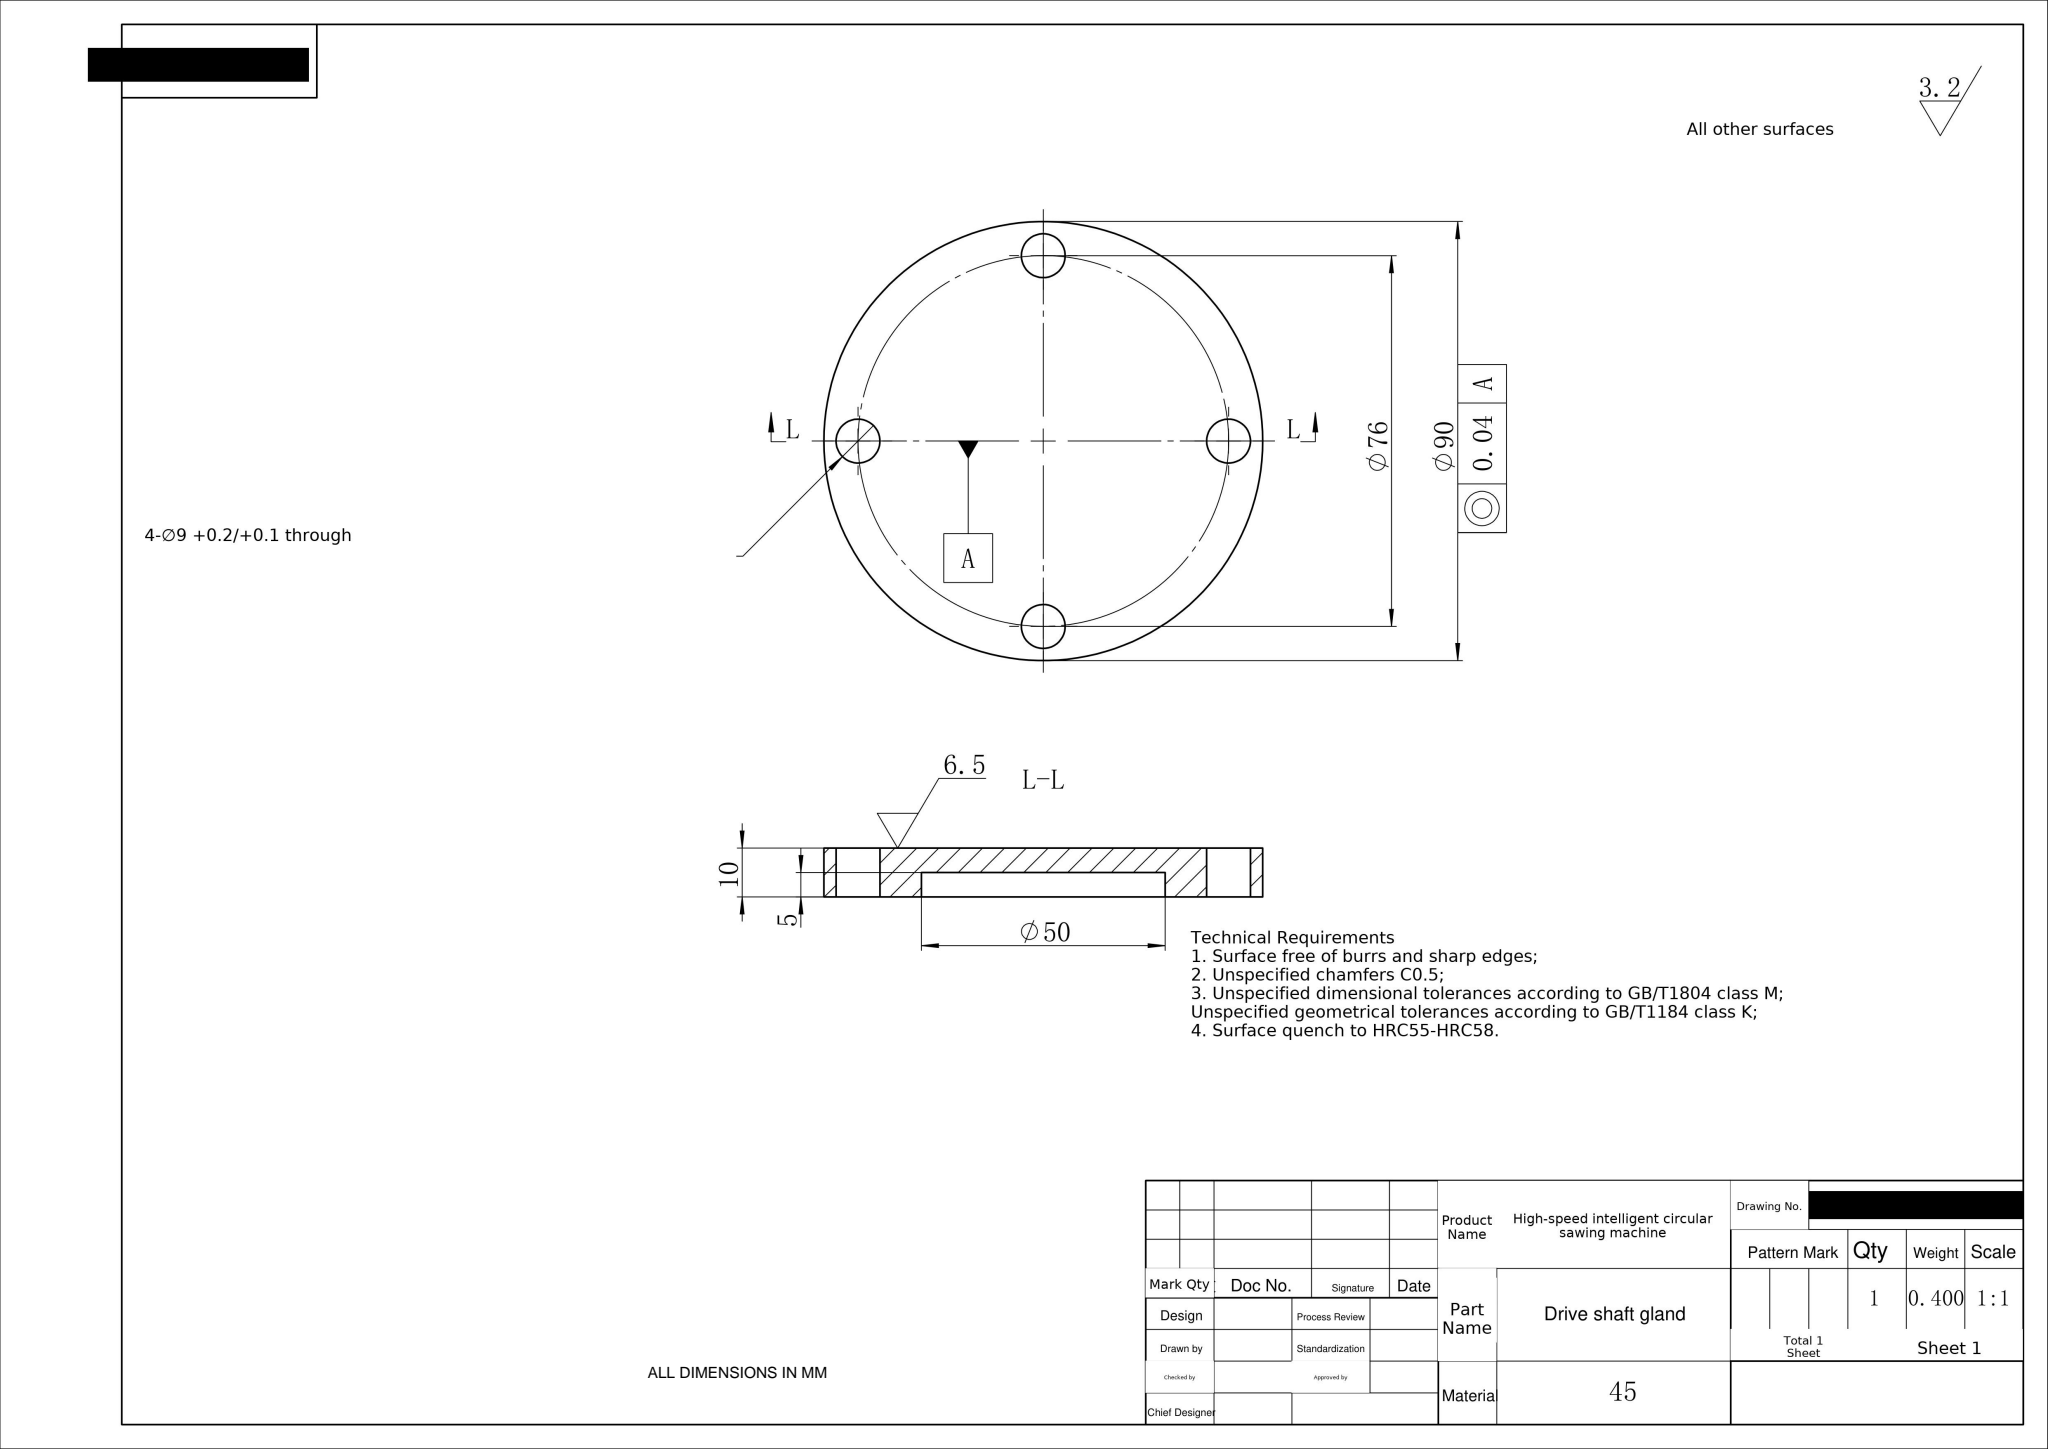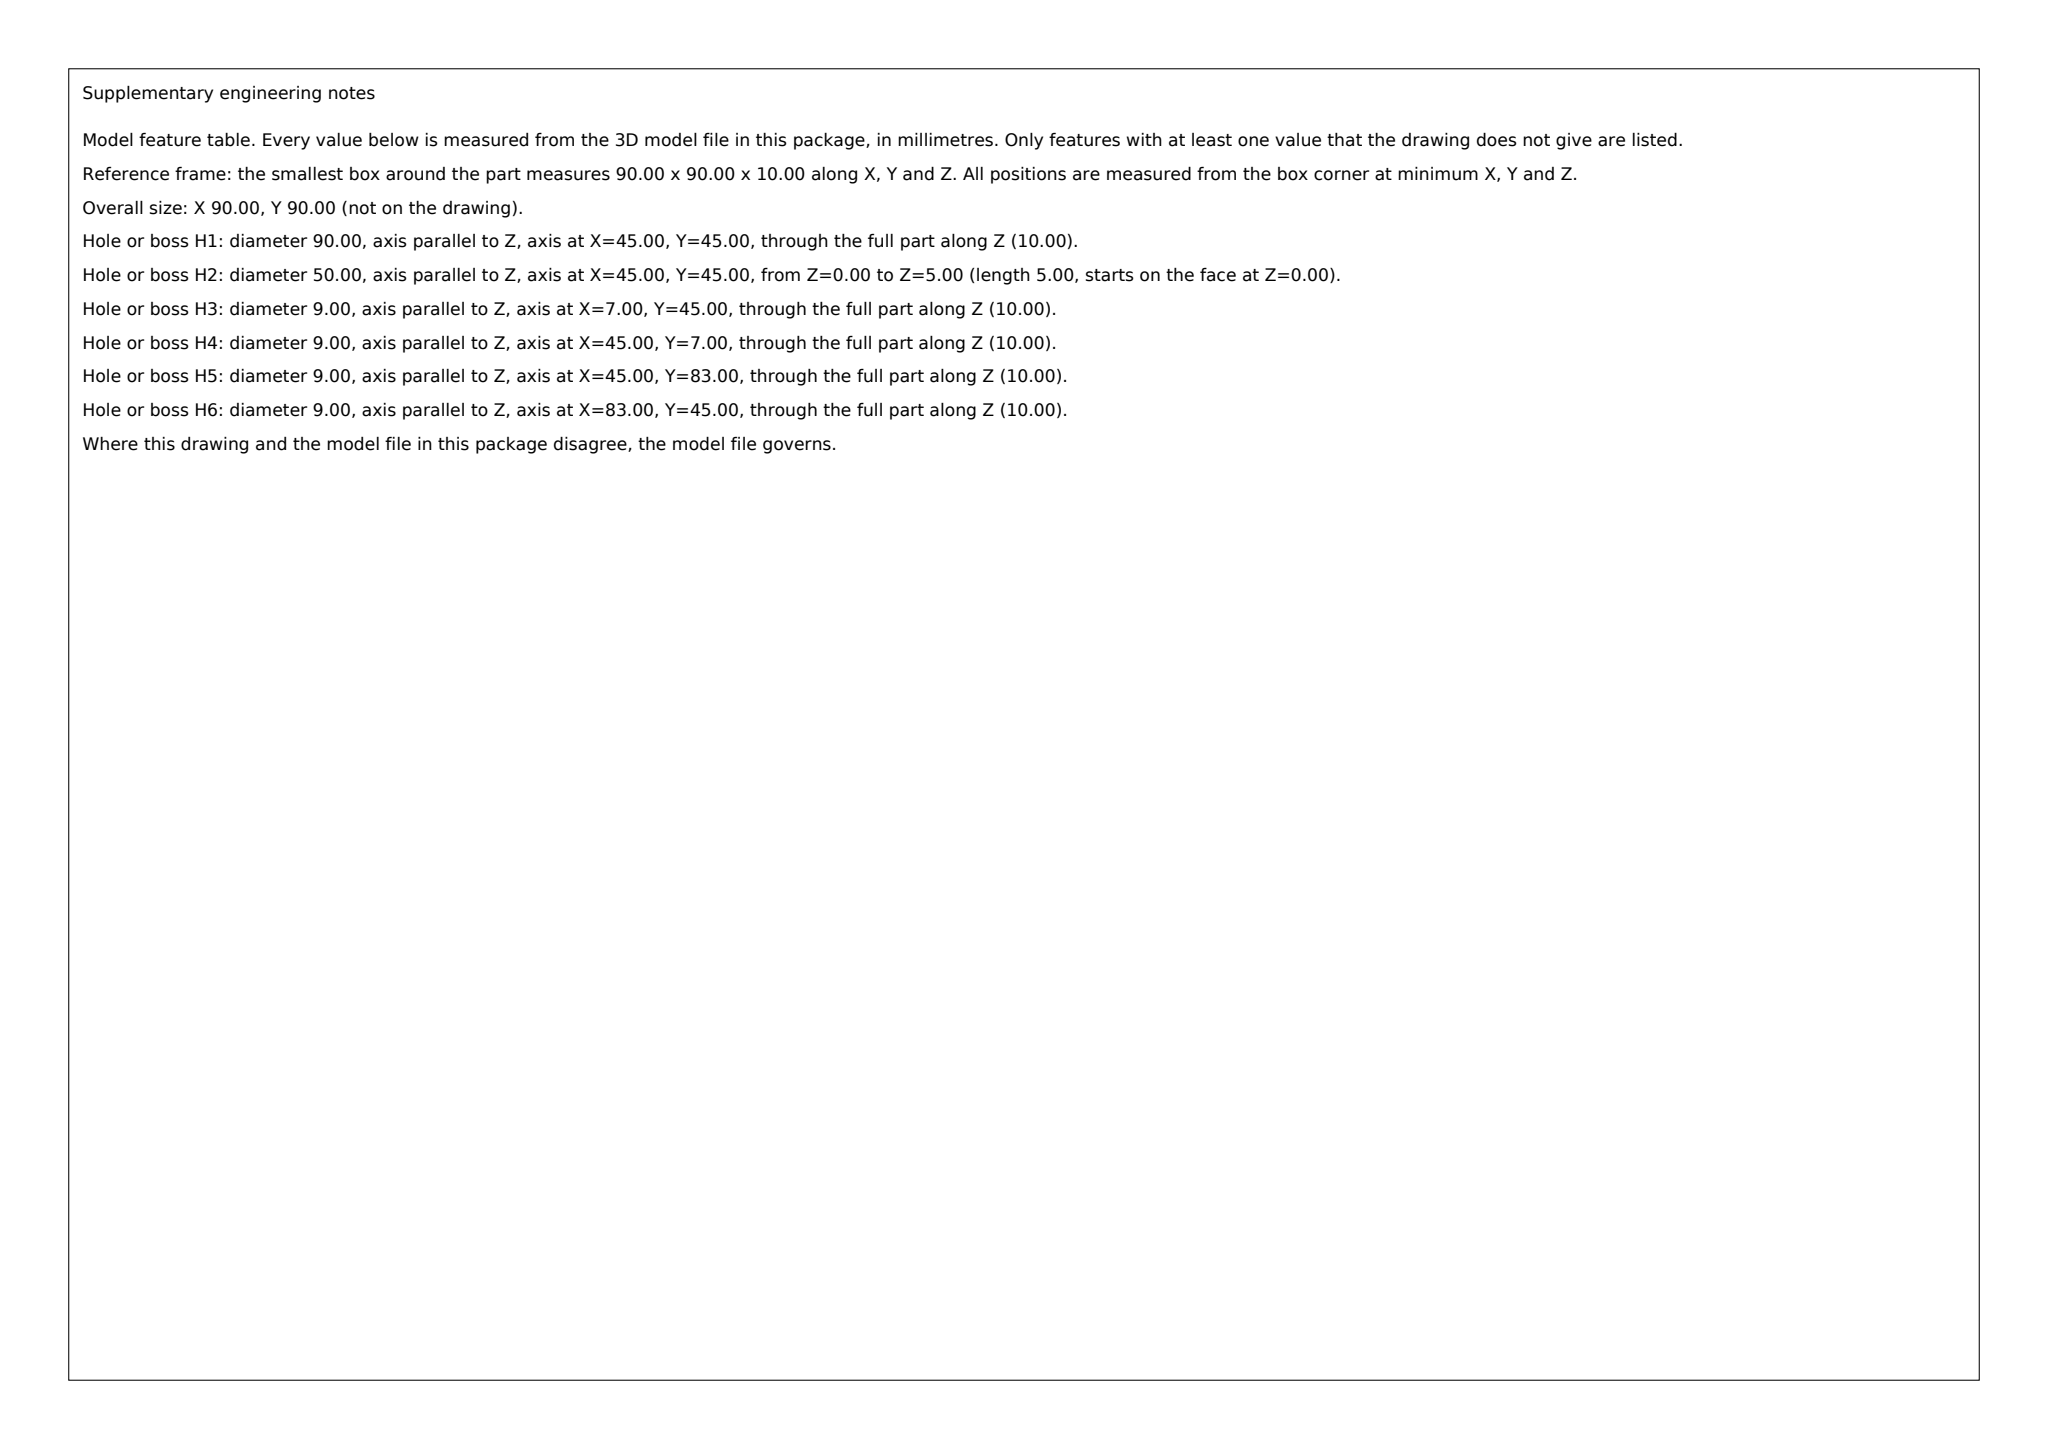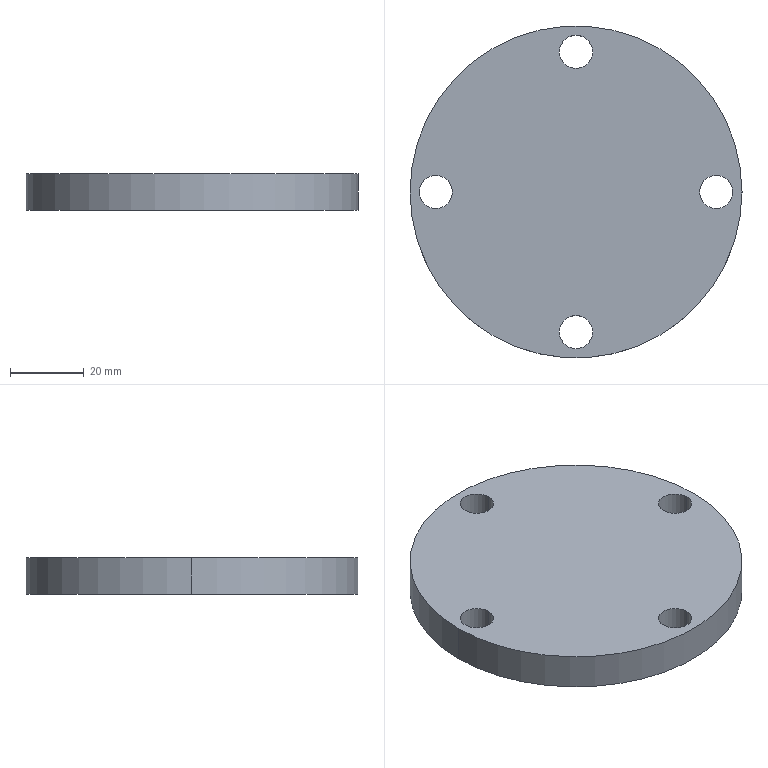Part | SolidWorks | mm | material 45 | 1 solid | 15 faces | box 90 x 90 x 10 mm | volume 51255 mm3 | cylinder 12 | plane 3 | commonest cylinder face diameters 9 x8 50 x2 90 x2
build123d program:
from build123d import *

# Parameters (mm, degrees)
SKETCH1_R           = 45
BOSS_EXTRUDE1_DEPTH = 10
SKETCH4_R           = 4.5
CUT_EXTRUDE2_DEPTH  = 65.42
SKETCH2_R           = 25
CUT_EXTRUDE3_DEPTH  = 5


with BuildPart() as part:
    # Sketch1 → Boss-Extrude1 (new body)
    with BuildSketch(Plane.XY):
        Circle(SKETCH1_R)
    extrude(amount=BOSS_EXTRUDE1_DEPTH)

    # Sketch4 → Cut-Extrude2 (cut, through all)
    with BuildSketch(Plane(origin=(0, 0, 0), x_dir=(-1, 0, 0), z_dir=(0, 0, -1))):
        with Locations((0, -38)):
            Circle(SKETCH4_R)
        with Locations((38, 0)):
            Circle(SKETCH4_R)
        with Locations((0, 38)):
            Circle(SKETCH4_R)
        with Locations((-38, 0)):
            Circle(SKETCH4_R)
    extrude(amount=-CUT_EXTRUDE2_DEPTH, mode=Mode.SUBTRACT)

    # Sketch2 → Cut-Extrude3 (cut)
    with BuildSketch(Plane(origin=(0, 0, 0), x_dir=(-1, 0, 0), z_dir=(0, 0, -1))):
        Circle(SKETCH2_R)
    extrude(amount=-CUT_EXTRUDE3_DEPTH, mode=Mode.SUBTRACT)


solid = part.part
STEP:
#1=CARTESIAN_POINT('',(25.,0.,5.));
#2=VERTEX_POINT('',#1);
#3=CARTESIAN_POINT('',(-25.,0.,5.));
#4=VERTEX_POINT('',#3);
#5=CARTESIAN_POINT('',(0.,0.,5.));
#6=DIRECTION('',(0.,0.,-1.));
#7=DIRECTION('',(-1.,0.,0.));
#8=AXIS2_PLACEMENT_3D('',#5,#6,#7);
#9=CIRCLE('',#8,25.);
#10=EDGE_CURVE('',#2,#4,#9,.T.);
#11=ORIENTED_EDGE('',*,*,#10,.F.);
#12=CARTESIAN_POINT('',(25.,0.,0.));
#13=VERTEX_POINT('',#12);
#14=CARTESIAN_POINT('',(25.,0.,5.));
#15=DIRECTION('',(0.,0.,-1.));
#16=VECTOR('',#15,1000.);
#17=LINE('',#14,#16);
#18=EDGE_CURVE('',#2,#13,#17,.T.);
#19=ORIENTED_EDGE('',*,*,#18,.T.);
#20=CARTESIAN_POINT('',(-25.,0.,0.));
#21=VERTEX_POINT('',#20);
#22=CARTESIAN_POINT('',(0.,0.,0.));
#23=DIRECTION('',(0.,0.,-1.));
#24=DIRECTION('',(-1.,0.,0.));
#25=AXIS2_PLACEMENT_3D('',#22,#23,#24);
#26=CIRCLE('',#25,25.);
#27=EDGE_CURVE('',#13,#21,#26,.T.);
#28=ORIENTED_EDGE('',*,*,#27,.T.);
#29=CARTESIAN_POINT('',(-25.,0.,5.));
#30=DIRECTION('',(0.,0.,-1.));
#31=VECTOR('',#30,1000.);
#32=LINE('',#29,#31);
#33=EDGE_CURVE('',#4,#21,#32,.T.);
#34=ORIENTED_EDGE('',*,*,#33,.F.);
#35=EDGE_LOOP('',(#11,#19,#28,#34));
#36=FACE_OUTER_BOUND('',#35,.T.);
#37=CARTESIAN_POINT('',(0.,0.,5.));
#38=DIRECTION('',(0.,0.,-1.));
#39=DIRECTION('',(-1.,0.,0.));
#40=AXIS2_PLACEMENT_3D('',#37,#38,#39);
#41=CYLINDRICAL_SURFACE('',#40,25.);
#42=ADVANCED_FACE('',(#36),#41,.F.);
#43=CARTESIAN_POINT('',(42.5,0.,10.));
#44=VERTEX_POINT('',#43);
#45=CARTESIAN_POINT('',(33.5,0.,10.));
#46=VERTEX_POINT('',#45);
#47=CARTESIAN_POINT('',(38.,0.,10.));
#48=DIRECTION('',(0.,0.,-1.));
#49=DIRECTION('',(-1.,0.,0.));
#50=AXIS2_PLACEMENT_3D('',#47,#48,#49);
#51=CIRCLE('',#50,4.5);
#52=EDGE_CURVE('',#44,#46,#51,.T.);
#53=ORIENTED_EDGE('',*,*,#52,.F.);
#54=CARTESIAN_POINT('',(42.5,0.,0.));
#55=VERTEX_POINT('',#54);
#56=CARTESIAN_POINT('',(42.5,0.,10.));
#57=DIRECTION('',(0.,0.,-1.));
#58=VECTOR('',#57,1000.);
#59=LINE('',#56,#58);
#60=EDGE_CURVE('',#44,#55,#59,.T.);
#61=ORIENTED_EDGE('',*,*,#60,.T.);
#62=CARTESIAN_POINT('',(33.5,0.,0.));
#63=VERTEX_POINT('',#62);
#64=CARTESIAN_POINT('',(38.,0.,0.));
#65=DIRECTION('',(0.,0.,-1.));
#66=DIRECTION('',(-1.,0.,0.));
#67=AXIS2_PLACEMENT_3D('',#64,#65,#66);
#68=CIRCLE('',#67,4.5);
#69=EDGE_CURVE('',#55,#63,#68,.T.);
#70=ORIENTED_EDGE('',*,*,#69,.T.);
#71=CARTESIAN_POINT('',(33.5,0.,10.));
#72=DIRECTION('',(0.,0.,-1.));
#73=VECTOR('',#72,1000.);
#74=LINE('',#71,#73);
#75=EDGE_CURVE('',#46,#63,#74,.T.);
#76=ORIENTED_EDGE('',*,*,#75,.F.);
#77=EDGE_LOOP('',(#53,#61,#70,#76));
#78=FACE_OUTER_BOUND('',#77,.T.);
#79=CARTESIAN_POINT('',(38.,0.,10.));
#80=DIRECTION('',(0.,0.,-1.));
#81=DIRECTION('',(-1.,0.,0.));
#82=AXIS2_PLACEMENT_3D('',#79,#80,#81);
#83=CYLINDRICAL_SURFACE('',#82,4.5);
#84=ADVANCED_FACE('',(#78),#83,.F.);
#85=CARTESIAN_POINT('',(4.5,38.,10.));
#86=VERTEX_POINT('',#85);
#87=CARTESIAN_POINT('',(-4.5,38.,10.));
#88=VERTEX_POINT('',#87);
#89=CARTESIAN_POINT('',(0.,38.,10.));
#90=DIRECTION('',(0.,0.,-1.));
#91=DIRECTION('',(-1.,0.,0.));
#92=AXIS2_PLACEMENT_3D('',#89,#90,#91);
#93=CIRCLE('',#92,4.5);
#94=EDGE_CURVE('',#86,#88,#93,.T.);
#95=ORIENTED_EDGE('',*,*,#94,.F.);
#96=CARTESIAN_POINT('',(4.5,38.,0.));
#97=VERTEX_POINT('',#96);
#98=CARTESIAN_POINT('',(4.5,38.,10.));
#99=DIRECTION('',(0.,0.,-1.));
#100=VECTOR('',#99,1000.);
#101=LINE('',#98,#100);
#102=EDGE_CURVE('',#86,#97,#101,.T.);
#103=ORIENTED_EDGE('',*,*,#102,.T.);
#104=CARTESIAN_POINT('',(-4.5,38.,0.));
#105=VERTEX_POINT('',#104);
#106=CARTESIAN_POINT('',(0.,38.,0.));
#107=DIRECTION('',(0.,0.,-1.));
#108=DIRECTION('',(-1.,0.,0.));
#109=AXIS2_PLACEMENT_3D('',#106,#107,#108);
#110=CIRCLE('',#109,4.5);
#111=EDGE_CURVE('',#97,#105,#110,.T.);
#112=ORIENTED_EDGE('',*,*,#111,.T.);
#113=CARTESIAN_POINT('',(-4.5,38.,10.));
#114=DIRECTION('',(0.,0.,-1.));
#115=VECTOR('',#114,1000.);
#116=LINE('',#113,#115);
#117=EDGE_CURVE('',#88,#105,#116,.T.);
#118=ORIENTED_EDGE('',*,*,#117,.F.);
#119=EDGE_LOOP('',(#95,#103,#112,#118));
#120=FACE_OUTER_BOUND('',#119,.T.);
#121=CARTESIAN_POINT('',(0.,38.,10.));
#122=DIRECTION('',(0.,0.,-1.));
#123=DIRECTION('',(-1.,0.,0.));
#124=AXIS2_PLACEMENT_3D('',#121,#122,#123);
#125=CYLINDRICAL_SURFACE('',#124,4.5);
#126=ADVANCED_FACE('',(#120),#125,.F.);
#127=CARTESIAN_POINT('',(-33.5,0.,10.));
#128=VERTEX_POINT('',#127);
#129=CARTESIAN_POINT('',(-42.5,0.,10.));
#130=VERTEX_POINT('',#129);
#131=CARTESIAN_POINT('',(-38.,0.,10.));
#132=DIRECTION('',(0.,0.,-1.));
#133=DIRECTION('',(-1.,0.,0.));
#134=AXIS2_PLACEMENT_3D('',#131,#132,#133);
#135=CIRCLE('',#134,4.5);
#136=EDGE_CURVE('',#128,#130,#135,.T.);
#137=ORIENTED_EDGE('',*,*,#136,.F.);
#138=CARTESIAN_POINT('',(-33.5,0.,0.));
#139=VERTEX_POINT('',#138);
#140=CARTESIAN_POINT('',(-33.5,0.,10.));
#141=DIRECTION('',(0.,0.,-1.));
#142=VECTOR('',#141,1000.);
#143=LINE('',#140,#142);
#144=EDGE_CURVE('',#128,#139,#143,.T.);
#145=ORIENTED_EDGE('',*,*,#144,.T.);
#146=CARTESIAN_POINT('',(-42.5,0.,0.));
#147=VERTEX_POINT('',#146);
#148=CARTESIAN_POINT('',(-38.,0.,0.));
#149=DIRECTION('',(0.,0.,-1.));
#150=DIRECTION('',(-1.,0.,0.));
#151=AXIS2_PLACEMENT_3D('',#148,#149,#150);
#152=CIRCLE('',#151,4.5);
#153=EDGE_CURVE('',#139,#147,#152,.T.);
#154=ORIENTED_EDGE('',*,*,#153,.T.);
#155=CARTESIAN_POINT('',(-42.5,0.,10.));
#156=DIRECTION('',(0.,0.,-1.));
#157=VECTOR('',#156,1000.);
#158=LINE('',#155,#157);
#159=EDGE_CURVE('',#130,#147,#158,.T.);
#160=ORIENTED_EDGE('',*,*,#159,.F.);
#161=EDGE_LOOP('',(#137,#145,#154,#160));
#162=FACE_OUTER_BOUND('',#161,.T.);
#163=CARTESIAN_POINT('',(-38.,0.,10.));
#164=DIRECTION('',(0.,0.,-1.));
#165=DIRECTION('',(-1.,0.,0.));
#166=AXIS2_PLACEMENT_3D('',#163,#164,#165);
#167=CYLINDRICAL_SURFACE('',#166,4.5);
#168=ADVANCED_FACE('',(#162),#167,.F.);
#169=CARTESIAN_POINT('',(4.5,-38.,10.));
#170=VERTEX_POINT('',#169);
#171=CARTESIAN_POINT('',(-4.5,-38.,10.));
#172=VERTEX_POINT('',#171);
#173=CARTESIAN_POINT('',(0.,-38.,10.));
#174=DIRECTION('',(0.,0.,-1.));
#175=DIRECTION('',(-1.,0.,0.));
#176=AXIS2_PLACEMENT_3D('',#173,#174,#175);
#177=CIRCLE('',#176,4.5);
#178=EDGE_CURVE('',#170,#172,#177,.T.);
#179=ORIENTED_EDGE('',*,*,#178,.F.);
#180=CARTESIAN_POINT('',(4.5,-38.,0.));
#181=VERTEX_POINT('',#180);
#182=CARTESIAN_POINT('',(4.5,-38.,10.));
#183=DIRECTION('',(0.,0.,-1.));
#184=VECTOR('',#183,1000.);
#185=LINE('',#182,#184);
#186=EDGE_CURVE('',#170,#181,#185,.T.);
#187=ORIENTED_EDGE('',*,*,#186,.T.);
#188=CARTESIAN_POINT('',(-4.5,-38.,0.));
#189=VERTEX_POINT('',#188);
#190=CARTESIAN_POINT('',(0.,-38.,0.));
#191=DIRECTION('',(0.,0.,-1.));
#192=DIRECTION('',(-1.,0.,0.));
#193=AXIS2_PLACEMENT_3D('',#190,#191,#192);
#194=CIRCLE('',#193,4.5);
#195=EDGE_CURVE('',#181,#189,#194,.T.);
#196=ORIENTED_EDGE('',*,*,#195,.T.);
#197=CARTESIAN_POINT('',(-4.5,-38.,10.));
#198=DIRECTION('',(0.,0.,-1.));
#199=VECTOR('',#198,1000.);
#200=LINE('',#197,#199);
#201=EDGE_CURVE('',#172,#189,#200,.T.);
#202=ORIENTED_EDGE('',*,*,#201,.F.);
#203=EDGE_LOOP('',(#179,#187,#196,#202));
#204=FACE_OUTER_BOUND('',#203,.T.);
#205=CARTESIAN_POINT('',(0.,-38.,10.));
#206=DIRECTION('',(0.,0.,-1.));
#207=DIRECTION('',(-1.,0.,0.));
#208=AXIS2_PLACEMENT_3D('',#205,#206,#207);
#209=CYLINDRICAL_SURFACE('',#208,4.5);
#210=ADVANCED_FACE('',(#204),#209,.F.);
#211=CARTESIAN_POINT('',(45.,0.,10.));
#212=VERTEX_POINT('',#211);
#213=CARTESIAN_POINT('',(-45.,0.,10.));
#214=VERTEX_POINT('',#213);
#215=CARTESIAN_POINT('',(0.,0.,10.));
#216=DIRECTION('',(0.,0.,1.));
#217=DIRECTION('',(1.,0.,0.));
#218=AXIS2_PLACEMENT_3D('',#215,#216,#217);
#219=CIRCLE('',#218,45.);
#220=EDGE_CURVE('',#212,#214,#219,.T.);
#221=ORIENTED_EDGE('',*,*,#220,.F.);
#222=CARTESIAN_POINT('',(45.,0.,0.));
#223=VERTEX_POINT('',#222);
#224=CARTESIAN_POINT('',(45.,0.,10.));
#225=DIRECTION('',(0.,0.,-1.));
#226=VECTOR('',#225,1000.);
#227=LINE('',#224,#226);
#228=EDGE_CURVE('',#212,#223,#227,.T.);
#229=ORIENTED_EDGE('',*,*,#228,.T.);
#230=CARTESIAN_POINT('',(-45.,0.,0.));
#231=VERTEX_POINT('',#230);
#232=CARTESIAN_POINT('',(0.,0.,0.));
#233=DIRECTION('',(0.,0.,1.));
#234=DIRECTION('',(1.,0.,0.));
#235=AXIS2_PLACEMENT_3D('',#232,#233,#234);
#236=CIRCLE('',#235,45.);
#237=EDGE_CURVE('',#223,#231,#236,.T.);
#238=ORIENTED_EDGE('',*,*,#237,.T.);
#239=CARTESIAN_POINT('',(-45.,0.,10.));
#240=DIRECTION('',(0.,0.,-1.));
#241=VECTOR('',#240,1000.);
#242=LINE('',#239,#241);
#243=EDGE_CURVE('',#214,#231,#242,.T.);
#244=ORIENTED_EDGE('',*,*,#243,.F.);
#245=EDGE_LOOP('',(#221,#229,#238,#244));
#246=FACE_OUTER_BOUND('',#245,.T.);
#247=CARTESIAN_POINT('',(0.,0.,10.));
#248=DIRECTION('',(0.,0.,-1.));
#249=DIRECTION('',(-1.,0.,0.));
#250=AXIS2_PLACEMENT_3D('',#247,#248,#249);
#251=CYLINDRICAL_SURFACE('',#250,45.);
#252=ADVANCED_FACE('',(#246),#251,.T.);
#253=ORIENTED_EDGE('',*,*,#228,.F.);
#254=CARTESIAN_POINT('',(0.,0.,10.));
#255=DIRECTION('',(0.,0.,1.));
#256=DIRECTION('',(1.,0.,0.));
#257=AXIS2_PLACEMENT_3D('',#254,#255,#256);
#258=CIRCLE('',#257,45.);
#259=EDGE_CURVE('',#214,#212,#258,.T.);
#260=ORIENTED_EDGE('',*,*,#259,.F.);
#261=ORIENTED_EDGE('',*,*,#243,.T.);
#262=CARTESIAN_POINT('',(0.,0.,0.));
#263=DIRECTION('',(0.,0.,1.));
#264=DIRECTION('',(1.,0.,0.));
#265=AXIS2_PLACEMENT_3D('',#262,#263,#264);
#266=CIRCLE('',#265,45.);
#267=EDGE_CURVE('',#231,#223,#266,.T.);
#268=ORIENTED_EDGE('',*,*,#267,.T.);
#269=EDGE_LOOP('',(#253,#260,#261,#268));
#270=FACE_OUTER_BOUND('',#269,.T.);
#271=CARTESIAN_POINT('',(0.,0.,10.));
#272=DIRECTION('',(0.,0.,-1.));
#273=DIRECTION('',(-1.,0.,0.));
#274=AXIS2_PLACEMENT_3D('',#271,#272,#273);
#275=CYLINDRICAL_SURFACE('',#274,45.);
#276=ADVANCED_FACE('',(#270),#275,.T.);
#277=CARTESIAN_POINT('',(38.,0.,10.));
#278=DIRECTION('',(0.,0.,-1.));
#279=DIRECTION('',(-1.,0.,0.));
#280=AXIS2_PLACEMENT_3D('',#277,#278,#279);
#281=CIRCLE('',#280,4.5);
#282=EDGE_CURVE('',#46,#44,#281,.T.);
#283=ORIENTED_EDGE('',*,*,#282,.T.);
#284=ORIENTED_EDGE('',*,*,#52,.T.);
#285=EDGE_LOOP('',(#283,#284));
#286=FACE_BOUND('',#285,.T.);
#287=CARTESIAN_POINT('',(0.,38.,10.));
#288=DIRECTION('',(0.,0.,-1.));
#289=DIRECTION('',(-1.,0.,0.));
#290=AXIS2_PLACEMENT_3D('',#287,#288,#289);
#291=CIRCLE('',#290,4.5);
#292=EDGE_CURVE('',#88,#86,#291,.T.);
#293=ORIENTED_EDGE('',*,*,#292,.T.);
#294=ORIENTED_EDGE('',*,*,#94,.T.);
#295=EDGE_LOOP('',(#293,#294));
#296=FACE_BOUND('',#295,.T.);
#297=CARTESIAN_POINT('',(-38.,0.,10.));
#298=DIRECTION('',(0.,0.,-1.));
#299=DIRECTION('',(-1.,0.,0.));
#300=AXIS2_PLACEMENT_3D('',#297,#298,#299);
#301=CIRCLE('',#300,4.5);
#302=EDGE_CURVE('',#130,#128,#301,.T.);
#303=ORIENTED_EDGE('',*,*,#302,.T.);
#304=ORIENTED_EDGE('',*,*,#136,.T.);
#305=EDGE_LOOP('',(#303,#304));
#306=FACE_BOUND('',#305,.T.);
#307=CARTESIAN_POINT('',(0.,-38.,10.));
#308=DIRECTION('',(0.,0.,-1.));
#309=DIRECTION('',(-1.,0.,0.));
#310=AXIS2_PLACEMENT_3D('',#307,#308,#309);
#311=CIRCLE('',#310,4.5);
#312=EDGE_CURVE('',#172,#170,#311,.T.);
#313=ORIENTED_EDGE('',*,*,#312,.T.);
#314=ORIENTED_EDGE('',*,*,#178,.T.);
#315=EDGE_LOOP('',(#313,#314));
#316=FACE_BOUND('',#315,.T.);
#317=ORIENTED_EDGE('',*,*,#259,.T.);
#318=ORIENTED_EDGE('',*,*,#220,.T.);
#319=EDGE_LOOP('',(#317,#318));
#320=FACE_OUTER_BOUND('',#319,.T.);
#321=CARTESIAN_POINT('',(0.,0.,10.));
#322=DIRECTION('',(0.,0.,1.));
#323=DIRECTION('',(1.,0.,0.));
#324=AXIS2_PLACEMENT_3D('',#321,#322,#323);
#325=PLANE('',#324);
#326=ADVANCED_FACE('',(#286,#296,#306,#316,#320),#325,.T.);
#327=CARTESIAN_POINT('',(0.,0.,0.));
#328=DIRECTION('',(0.,0.,-1.));
#329=DIRECTION('',(-1.,0.,0.));
#330=AXIS2_PLACEMENT_3D('',#327,#328,#329);
#331=CIRCLE('',#330,25.);
#332=EDGE_CURVE('',#21,#13,#331,.T.);
#333=ORIENTED_EDGE('',*,*,#332,.F.);
#334=ORIENTED_EDGE('',*,*,#27,.F.);
#335=EDGE_LOOP('',(#333,#334));
#336=FACE_BOUND('',#335,.T.);
#337=CARTESIAN_POINT('',(38.,0.,0.));
#338=DIRECTION('',(0.,0.,-1.));
#339=DIRECTION('',(-1.,0.,0.));
#340=AXIS2_PLACEMENT_3D('',#337,#338,#339);
#341=CIRCLE('',#340,4.5);
#342=EDGE_CURVE('',#63,#55,#341,.T.);
#343=ORIENTED_EDGE('',*,*,#342,.F.);
#344=ORIENTED_EDGE('',*,*,#69,.F.);
#345=EDGE_LOOP('',(#343,#344));
#346=FACE_BOUND('',#345,.T.);
#347=CARTESIAN_POINT('',(0.,38.,0.));
#348=DIRECTION('',(0.,0.,-1.));
#349=DIRECTION('',(-1.,0.,0.));
#350=AXIS2_PLACEMENT_3D('',#347,#348,#349);
#351=CIRCLE('',#350,4.5);
#352=EDGE_CURVE('',#105,#97,#351,.T.);
#353=ORIENTED_EDGE('',*,*,#352,.F.);
#354=ORIENTED_EDGE('',*,*,#111,.F.);
#355=EDGE_LOOP('',(#353,#354));
#356=FACE_BOUND('',#355,.T.);
#357=CARTESIAN_POINT('',(-38.,0.,0.));
#358=DIRECTION('',(0.,0.,-1.));
#359=DIRECTION('',(-1.,0.,0.));
#360=AXIS2_PLACEMENT_3D('',#357,#358,#359);
#361=CIRCLE('',#360,4.5);
#362=EDGE_CURVE('',#147,#139,#361,.T.);
#363=ORIENTED_EDGE('',*,*,#362,.F.);
#364=ORIENTED_EDGE('',*,*,#153,.F.);
#365=EDGE_LOOP('',(#363,#364));
#366=FACE_BOUND('',#365,.T.);
#367=CARTESIAN_POINT('',(0.,-38.,0.));
#368=DIRECTION('',(0.,0.,-1.));
#369=DIRECTION('',(-1.,0.,0.));
#370=AXIS2_PLACEMENT_3D('',#367,#368,#369);
#371=CIRCLE('',#370,4.5);
#372=EDGE_CURVE('',#189,#181,#371,.T.);
#373=ORIENTED_EDGE('',*,*,#372,.F.);
#374=ORIENTED_EDGE('',*,*,#195,.F.);
#375=EDGE_LOOP('',(#373,#374));
#376=FACE_BOUND('',#375,.T.);
#377=ORIENTED_EDGE('',*,*,#267,.F.);
#378=ORIENTED_EDGE('',*,*,#237,.F.);
#379=EDGE_LOOP('',(#377,#378));
#380=FACE_OUTER_BOUND('',#379,.T.);
#381=CARTESIAN_POINT('',(0.,0.,0.));
#382=DIRECTION('',(0.,0.,1.));
#383=DIRECTION('',(1.,0.,0.));
#384=AXIS2_PLACEMENT_3D('',#381,#382,#383);
#385=PLANE('',#384);
#386=ADVANCED_FACE('',(#336,#346,#356,#366,#376,#380),#385,.F.);
#387=ORIENTED_EDGE('',*,*,#186,.F.);
#388=ORIENTED_EDGE('',*,*,#312,.F.);
#389=ORIENTED_EDGE('',*,*,#201,.T.);
#390=ORIENTED_EDGE('',*,*,#372,.T.);
#391=EDGE_LOOP('',(#387,#388,#389,#390));
#392=FACE_OUTER_BOUND('',#391,.T.);
#393=CARTESIAN_POINT('',(0.,-38.,10.));
#394=DIRECTION('',(0.,0.,-1.));
#395=DIRECTION('',(-1.,0.,0.));
#396=AXIS2_PLACEMENT_3D('',#393,#394,#395);
#397=CYLINDRICAL_SURFACE('',#396,4.5);
#398=ADVANCED_FACE('',(#392),#397,.F.);
#399=ORIENTED_EDGE('',*,*,#144,.F.);
#400=ORIENTED_EDGE('',*,*,#302,.F.);
#401=ORIENTED_EDGE('',*,*,#159,.T.);
#402=ORIENTED_EDGE('',*,*,#362,.T.);
#403=EDGE_LOOP('',(#399,#400,#401,#402));
#404=FACE_OUTER_BOUND('',#403,.T.);
#405=CARTESIAN_POINT('',(-38.,0.,10.));
#406=DIRECTION('',(0.,0.,-1.));
#407=DIRECTION('',(-1.,0.,0.));
#408=AXIS2_PLACEMENT_3D('',#405,#406,#407);
#409=CYLINDRICAL_SURFACE('',#408,4.5);
#410=ADVANCED_FACE('',(#404),#409,.F.);
#411=ORIENTED_EDGE('',*,*,#102,.F.);
#412=ORIENTED_EDGE('',*,*,#292,.F.);
#413=ORIENTED_EDGE('',*,*,#117,.T.);
#414=ORIENTED_EDGE('',*,*,#352,.T.);
#415=EDGE_LOOP('',(#411,#412,#413,#414));
#416=FACE_OUTER_BOUND('',#415,.T.);
#417=CARTESIAN_POINT('',(0.,38.,10.));
#418=DIRECTION('',(0.,0.,-1.));
#419=DIRECTION('',(-1.,0.,0.));
#420=AXIS2_PLACEMENT_3D('',#417,#418,#419);
#421=CYLINDRICAL_SURFACE('',#420,4.5);
#422=ADVANCED_FACE('',(#416),#421,.F.);
#423=ORIENTED_EDGE('',*,*,#60,.F.);
#424=ORIENTED_EDGE('',*,*,#282,.F.);
#425=ORIENTED_EDGE('',*,*,#75,.T.);
#426=ORIENTED_EDGE('',*,*,#342,.T.);
#427=EDGE_LOOP('',(#423,#424,#425,#426));
#428=FACE_OUTER_BOUND('',#427,.T.);
#429=CARTESIAN_POINT('',(38.,0.,10.));
#430=DIRECTION('',(0.,0.,-1.));
#431=DIRECTION('',(-1.,0.,0.));
#432=AXIS2_PLACEMENT_3D('',#429,#430,#431);
#433=CYLINDRICAL_SURFACE('',#432,4.5);
#434=ADVANCED_FACE('',(#428),#433,.F.);
#435=ORIENTED_EDGE('',*,*,#18,.F.);
#436=CARTESIAN_POINT('',(0.,0.,5.));
#437=DIRECTION('',(0.,0.,-1.));
#438=DIRECTION('',(-1.,0.,0.));
#439=AXIS2_PLACEMENT_3D('',#436,#437,#438);
#440=CIRCLE('',#439,25.);
#441=EDGE_CURVE('',#4,#2,#440,.T.);
#442=ORIENTED_EDGE('',*,*,#441,.F.);
#443=ORIENTED_EDGE('',*,*,#33,.T.);
#444=ORIENTED_EDGE('',*,*,#332,.T.);
#445=EDGE_LOOP('',(#435,#442,#443,#444));
#446=FACE_OUTER_BOUND('',#445,.T.);
#447=CARTESIAN_POINT('',(0.,0.,5.));
#448=DIRECTION('',(0.,0.,-1.));
#449=DIRECTION('',(-1.,0.,0.));
#450=AXIS2_PLACEMENT_3D('',#447,#448,#449);
#451=CYLINDRICAL_SURFACE('',#450,25.);
#452=ADVANCED_FACE('',(#446),#451,.F.);
#453=ORIENTED_EDGE('',*,*,#441,.T.);
#454=ORIENTED_EDGE('',*,*,#10,.T.);
#455=EDGE_LOOP('',(#453,#454));
#456=FACE_OUTER_BOUND('',#455,.T.);
#457=CARTESIAN_POINT('',(0.,0.,5.));
#458=DIRECTION('',(0.,0.,-1.));
#459=DIRECTION('',(-1.,0.,0.));
#460=AXIS2_PLACEMENT_3D('',#457,#458,#459);
#461=PLANE('',#460);
#462=ADVANCED_FACE('',(#456),#461,.T.);
#463=CLOSED_SHELL('',(#42,#84,#126,#168,#210,#252,#276,#326,#386,#398,#410,#422,#434,#452,#462));
#464=MANIFOLD_SOLID_BREP('',#463);
#465=CARTESIAN_POINT('',(0.,0.,0.));
#466=DIRECTION('',(0.,0.,1.));
#467=DIRECTION('',(1.,0.,0.));
#468=AXIS2_PLACEMENT_3D('',#465,#466,#467);
#469=(LENGTH_UNIT()NAMED_UNIT(*)SI_UNIT(.MILLI.,.METRE.));
#470=UNCERTAINTY_MEASURE_WITH_UNIT(LENGTH_MEASURE(0.00001),#469,'','');
#471=(NAMED_UNIT(*)PLANE_ANGLE_UNIT()SI_UNIT($,.RADIAN.));
#472=(NAMED_UNIT(*)SI_UNIT($,.STERADIAN.)SOLID_ANGLE_UNIT());
#473=(GEOMETRIC_REPRESENTATION_CONTEXT(3)GLOBAL_UNCERTAINTY_ASSIGNED_CONTEXT((#470))GLOBAL_UNIT_ASSIGNED_CONTEXT((#469,#471,#472))REPRESENTATION_CONTEXT('',''));
#474=ADVANCED_BREP_SHAPE_REPRESENTATION('',(#464,#468),#473);